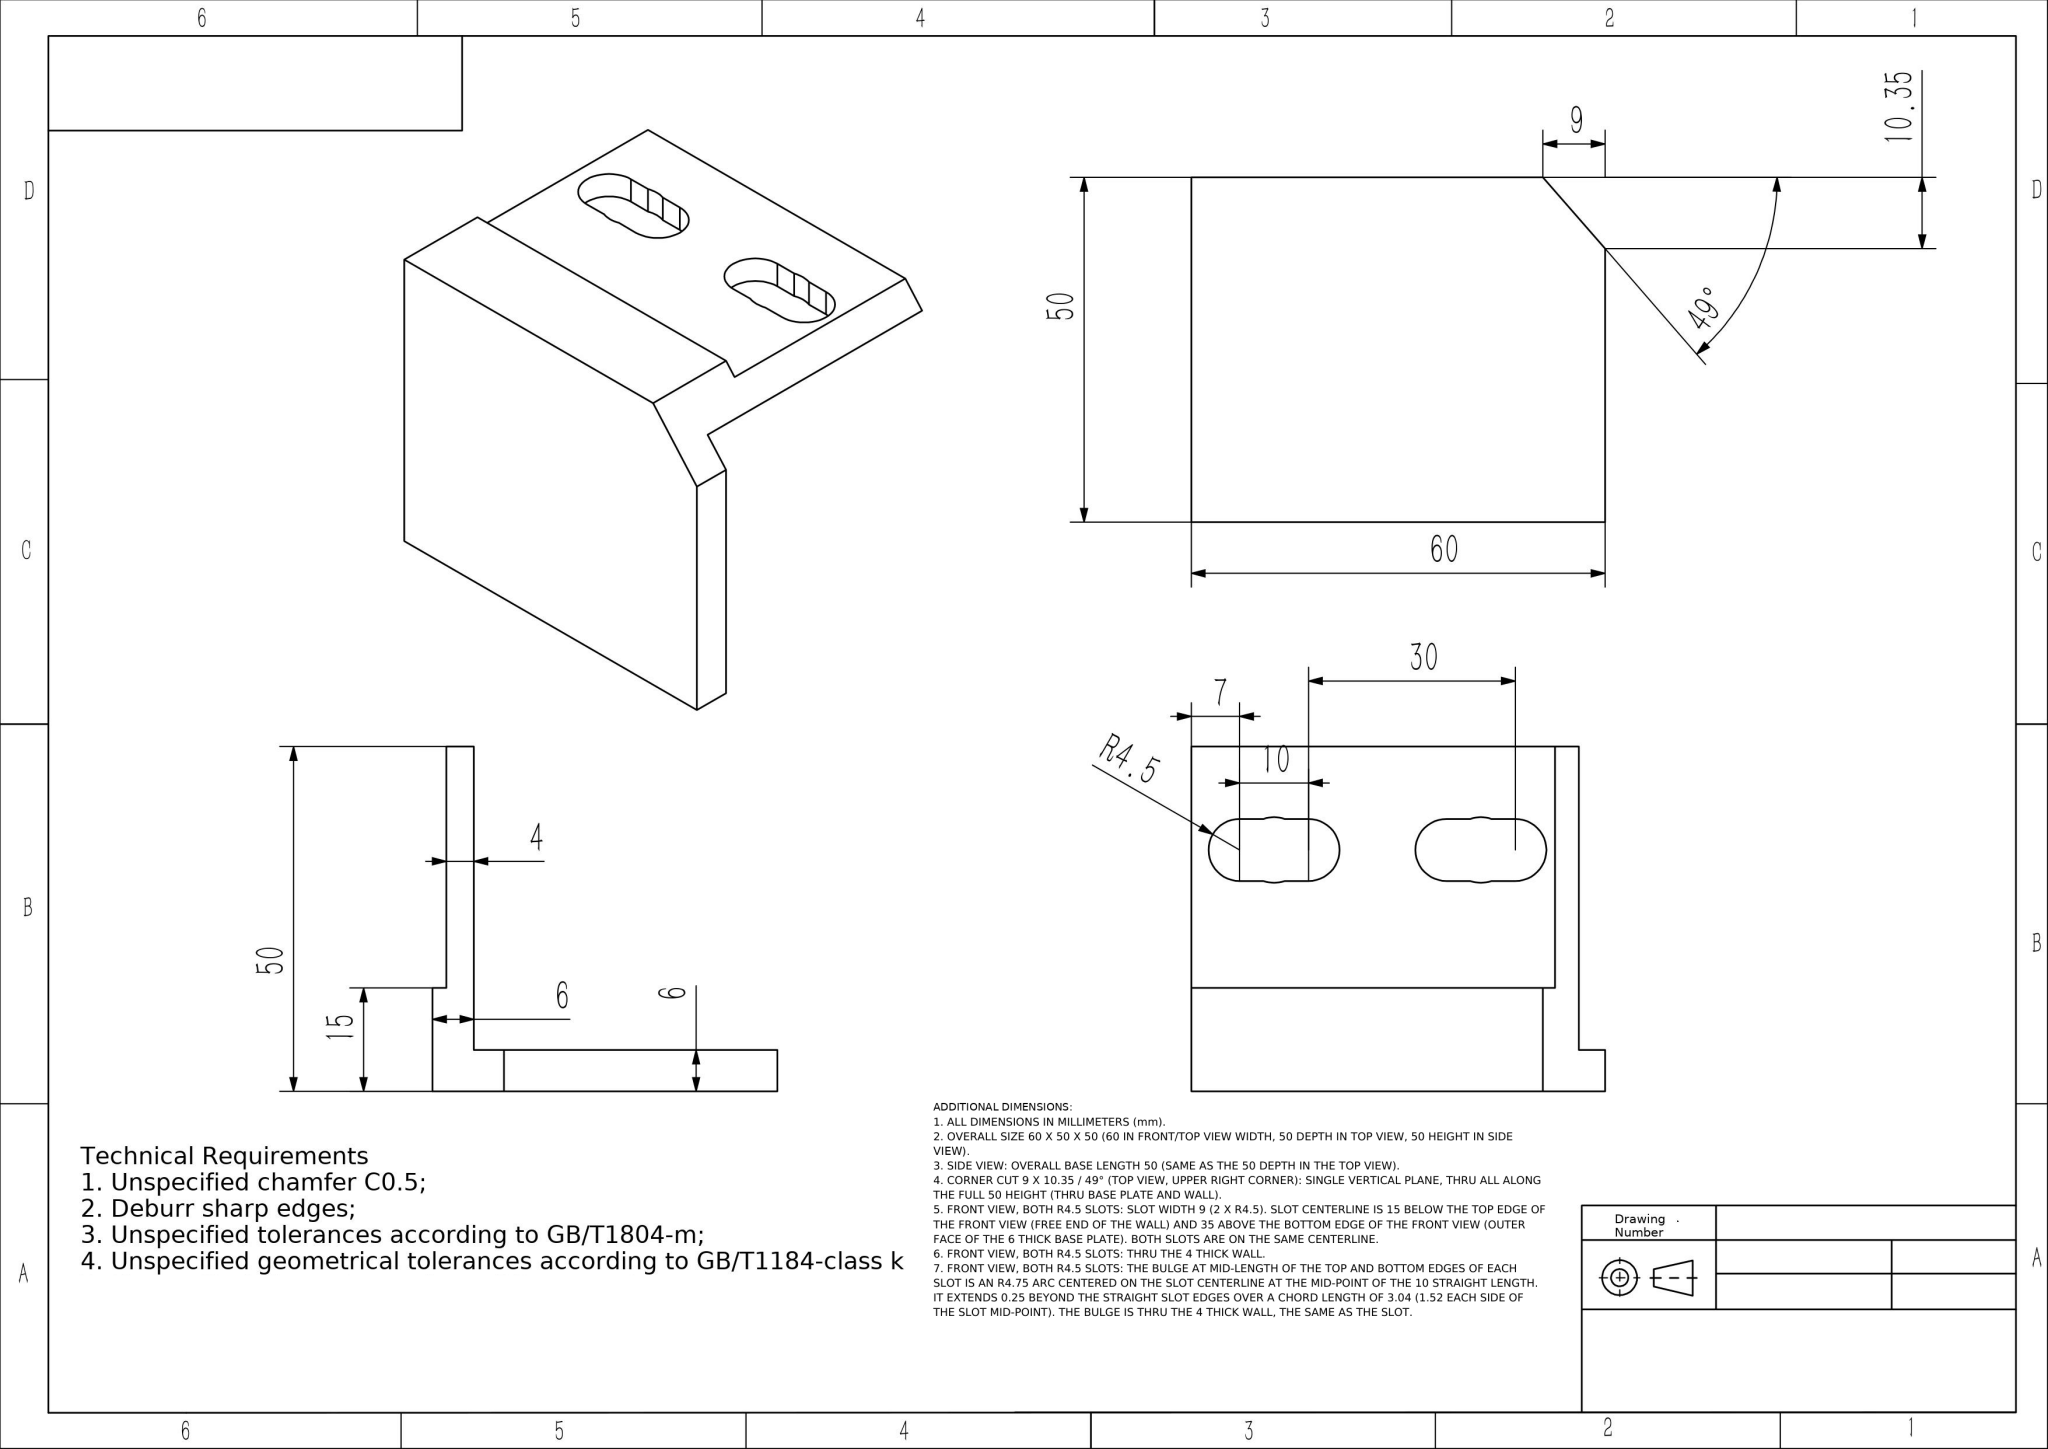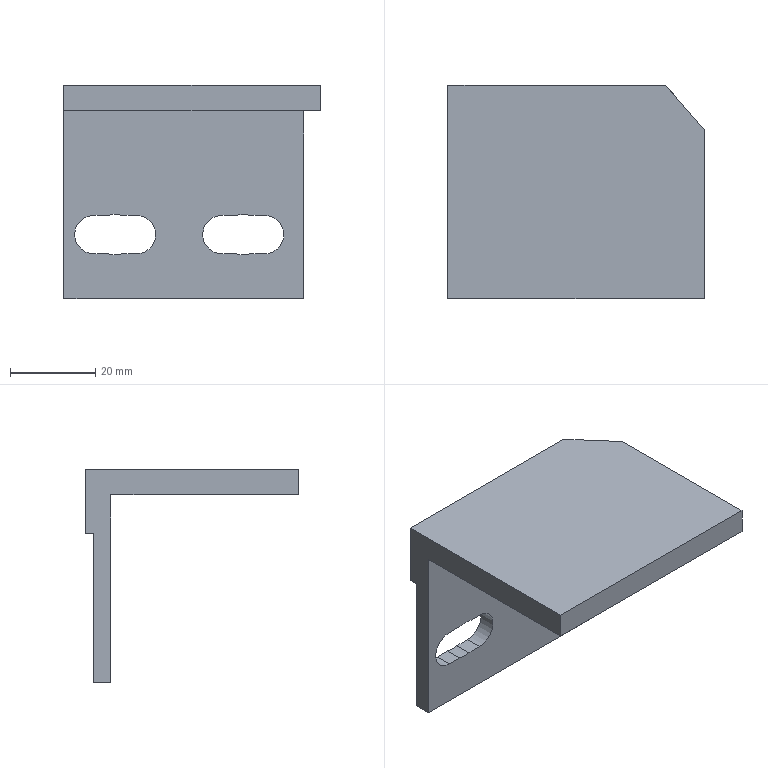Part | NX | mm | 1 solid | 29 faces | box 60 x 50 x 50 mm | volume 27005 mm3 | plane 19 | cylinder 10 | commonest cylinder face diameters 9.5 x6 9 x4
STEP:
#1=COLOUR_RGB('',1.,0.,1.);
#2=FILL_AREA_STYLE_COLOUR('',#1);
#3=FILL_AREA_STYLE('',(#2));
#4=SURFACE_STYLE_FILL_AREA(#3);
#5=SURFACE_SIDE_STYLE('',(#4));
#6=SURFACE_STYLE_USAGE(.BOTH.,#5);
#7=PRESENTATION_STYLE_ASSIGNMENT((#6));
#8=CARTESIAN_POINT('',(12.,19.,-24.25));
#9=VERTEX_POINT('',#8);
#10=CARTESIAN_POINT('',(13.521,19.,-24.5));
#11=VERTEX_POINT('',#10);
#12=CARTESIAN_POINT('',(12.,19.,-29.));
#13=DIRECTION('',(0.,1.,0.));
#14=DIRECTION('',(0.,0.,1.));
#15=AXIS2_PLACEMENT_3D('',#12,#13,#14);
#16=CIRCLE('',#15,4.75);
#17=EDGE_CURVE('',#9,#11,#16,.T.);
#18=ORIENTED_EDGE('',*,*,#17,.F.);
#19=CARTESIAN_POINT('',(12.,23.,-24.25));
#20=VERTEX_POINT('',#19);
#21=CARTESIAN_POINT('',(12.,23.,-24.25));
#22=DIRECTION('',(0.,1.,0.));
#23=VECTOR('',#22,1000.);
#24=LINE('',#21,#23);
#25=EDGE_CURVE('',#9,#20,#24,.T.);
#26=ORIENTED_EDGE('',*,*,#25,.T.);
#27=CARTESIAN_POINT('',(13.521,23.,-24.5));
#28=VERTEX_POINT('',#27);
#29=CARTESIAN_POINT('',(12.,23.,-29.));
#30=DIRECTION('',(0.,1.,0.));
#31=DIRECTION('',(0.,0.,1.));
#32=AXIS2_PLACEMENT_3D('',#29,#30,#31);
#33=CIRCLE('',#32,4.75);
#34=EDGE_CURVE('',#20,#28,#33,.T.);
#35=ORIENTED_EDGE('',*,*,#34,.T.);
#36=CARTESIAN_POINT('',(13.521,23.,-24.5));
#37=DIRECTION('',(0.,1.,0.));
#38=VECTOR('',#37,1000.);
#39=LINE('',#36,#38);
#40=EDGE_CURVE('',#11,#28,#39,.T.);
#41=ORIENTED_EDGE('',*,*,#40,.F.);
#42=EDGE_LOOP('',(#18,#26,#35,#41));
#43=FACE_OUTER_BOUND('',#42,.T.);
#44=CARTESIAN_POINT('',(12.,23.,-29.));
#45=DIRECTION('',(0.,1.,0.));
#46=DIRECTION('',(0.,0.,1.));
#47=AXIS2_PLACEMENT_3D('',#44,#45,#46);
#48=CYLINDRICAL_SURFACE('',#47,4.75);
#49=ADVANCED_FACE('',(#43),#48,.F.);
#50=CARTESIAN_POINT('',(-18.,19.,-24.25));
#51=VERTEX_POINT('',#50);
#52=CARTESIAN_POINT('',(-16.479,19.,-24.5));
#53=VERTEX_POINT('',#52);
#54=CARTESIAN_POINT('',(-18.,19.,-29.));
#55=DIRECTION('',(0.,1.,0.));
#56=DIRECTION('',(0.,0.,1.));
#57=AXIS2_PLACEMENT_3D('',#54,#55,#56);
#58=CIRCLE('',#57,4.75);
#59=EDGE_CURVE('',#51,#53,#58,.T.);
#60=ORIENTED_EDGE('',*,*,#59,.F.);
#61=CARTESIAN_POINT('',(-18.,23.,-24.25));
#62=VERTEX_POINT('',#61);
#63=CARTESIAN_POINT('',(-18.,23.,-24.25));
#64=DIRECTION('',(0.,1.,0.));
#65=VECTOR('',#64,1000.);
#66=LINE('',#63,#65);
#67=EDGE_CURVE('',#51,#62,#66,.T.);
#68=ORIENTED_EDGE('',*,*,#67,.T.);
#69=CARTESIAN_POINT('',(-16.479,23.,-24.5));
#70=VERTEX_POINT('',#69);
#71=CARTESIAN_POINT('',(-18.,23.,-29.));
#72=DIRECTION('',(0.,1.,0.));
#73=DIRECTION('',(0.,0.,1.));
#74=AXIS2_PLACEMENT_3D('',#71,#72,#73);
#75=CIRCLE('',#74,4.75);
#76=EDGE_CURVE('',#62,#70,#75,.T.);
#77=ORIENTED_EDGE('',*,*,#76,.T.);
#78=CARTESIAN_POINT('',(-16.479,23.,-24.5));
#79=DIRECTION('',(0.,1.,0.));
#80=VECTOR('',#79,1000.);
#81=LINE('',#78,#80);
#82=EDGE_CURVE('',#53,#70,#81,.T.);
#83=ORIENTED_EDGE('',*,*,#82,.F.);
#84=EDGE_LOOP('',(#60,#68,#77,#83));
#85=FACE_OUTER_BOUND('',#84,.T.);
#86=CARTESIAN_POINT('',(-18.,23.,-29.));
#87=DIRECTION('',(0.,1.,0.));
#88=DIRECTION('',(0.,0.,1.));
#89=AXIS2_PLACEMENT_3D('',#86,#87,#88);
#90=CYLINDRICAL_SURFACE('',#89,4.75);
#91=ADVANCED_FACE('',(#85),#90,.F.);
#92=CARTESIAN_POINT('',(10.479,19.,-33.5));
#93=VERTEX_POINT('',#92);
#94=CARTESIAN_POINT('',(7.,19.,-33.5));
#95=VERTEX_POINT('',#94);
#96=CARTESIAN_POINT('',(30.,19.,-33.5));
#97=DIRECTION('',(-1.,0.,0.));
#98=VECTOR('',#97,1000.);
#99=LINE('',#96,#98);
#100=EDGE_CURVE('',#93,#95,#99,.T.);
#101=ORIENTED_EDGE('',*,*,#100,.F.);
#102=CARTESIAN_POINT('',(10.479,23.,-33.5));
#103=VERTEX_POINT('',#102);
#104=CARTESIAN_POINT('',(10.479,23.,-33.5));
#105=DIRECTION('',(0.,1.,0.));
#106=VECTOR('',#105,1000.);
#107=LINE('',#104,#106);
#108=EDGE_CURVE('',#93,#103,#107,.T.);
#109=ORIENTED_EDGE('',*,*,#108,.T.);
#110=CARTESIAN_POINT('',(7.,23.,-33.5));
#111=VERTEX_POINT('',#110);
#112=CARTESIAN_POINT('',(7.,23.,-33.5));
#113=DIRECTION('',(-1.,0.,0.));
#114=VECTOR('',#113,1000.);
#115=LINE('',#112,#114);
#116=EDGE_CURVE('',#103,#111,#115,.T.);
#117=ORIENTED_EDGE('',*,*,#116,.T.);
#118=CARTESIAN_POINT('',(7.,-21.,-33.5));
#119=DIRECTION('',(0.,1.,0.));
#120=VECTOR('',#119,1000.);
#121=LINE('',#118,#120);
#122=EDGE_CURVE('',#95,#111,#121,.T.);
#123=ORIENTED_EDGE('',*,*,#122,.F.);
#124=EDGE_LOOP('',(#101,#109,#117,#123));
#125=FACE_OUTER_BOUND('',#124,.T.);
#126=CARTESIAN_POINT('',(7.,-21.,-33.5));
#127=DIRECTION('',(0.,0.,-1.));
#128=DIRECTION('',(0.,1.,0.));
#129=AXIS2_PLACEMENT_3D('',#126,#127,#128);
#130=PLANE('',#129);
#131=ADVANCED_FACE('',(#125),#130,.F.);
#132=CARTESIAN_POINT('',(-30.,23.,-9.));
#133=VERTEX_POINT('',#132);
#134=CARTESIAN_POINT('',(22.739,23.,-9.));
#135=VERTEX_POINT('',#134);
#136=CARTESIAN_POINT('',(-30.,23.,-9.));
#137=DIRECTION('',(1.,0.,0.));
#138=VECTOR('',#137,1000.);
#139=LINE('',#136,#138);
#140=EDGE_CURVE('',#133,#135,#139,.T.);
#141=ORIENTED_EDGE('',*,*,#140,.T.);
#142=CARTESIAN_POINT('',(22.739,23.,-44.));
#143=VERTEX_POINT('',#142);
#144=CARTESIAN_POINT('',(22.739,23.,-44.));
#145=DIRECTION('',(-0.,0.,-1.));
#146=VECTOR('',#145,1000.);
#147=LINE('',#144,#146);
#148=EDGE_CURVE('',#135,#143,#147,.T.);
#149=ORIENTED_EDGE('',*,*,#148,.T.);
#150=CARTESIAN_POINT('',(-30.,23.,-44.));
#151=VERTEX_POINT('',#150);
#152=CARTESIAN_POINT('',(0.,23.,-44.));
#153=DIRECTION('',(-1.,0.,0.));
#154=VECTOR('',#153,1000.);
#155=LINE('',#152,#154);
#156=EDGE_CURVE('',#143,#151,#155,.T.);
#157=ORIENTED_EDGE('',*,*,#156,.T.);
#158=CARTESIAN_POINT('',(-30.,23.,6.));
#159=DIRECTION('',(0.,0.,-1.));
#160=VECTOR('',#159,1000.);
#161=LINE('',#158,#160);
#162=EDGE_CURVE('',#133,#151,#161,.T.);
#163=ORIENTED_EDGE('',*,*,#162,.F.);
#164=EDGE_LOOP('',(#141,#149,#157,#163));
#165=FACE_OUTER_BOUND('',#164,.T.);
#166=CARTESIAN_POINT('',(-16.479,23.,-33.5));
#167=VERTEX_POINT('',#166);
#168=CARTESIAN_POINT('',(-19.521,23.,-33.5));
#169=VERTEX_POINT('',#168);
#170=CARTESIAN_POINT('',(-18.,23.,-29.));
#171=DIRECTION('',(0.,1.,0.));
#172=DIRECTION('',(0.,0.,1.));
#173=AXIS2_PLACEMENT_3D('',#170,#171,#172);
#174=CIRCLE('',#173,4.75);
#175=EDGE_CURVE('',#167,#169,#174,.T.);
#176=ORIENTED_EDGE('',*,*,#175,.F.);
#177=CARTESIAN_POINT('',(-13.,23.,-33.5));
#178=VERTEX_POINT('',#177);
#179=CARTESIAN_POINT('',(-23.,23.,-33.5));
#180=DIRECTION('',(-1.,0.,0.));
#181=VECTOR('',#180,1000.);
#182=LINE('',#179,#181);
#183=EDGE_CURVE('',#178,#167,#182,.T.);
#184=ORIENTED_EDGE('',*,*,#183,.F.);
#185=CARTESIAN_POINT('',(-13.,23.,-24.5));
#186=VERTEX_POINT('',#185);
#187=CARTESIAN_POINT('',(-13.,23.,-29.));
#188=DIRECTION('',(0.,1.,0.));
#189=DIRECTION('',(0.,0.,1.));
#190=AXIS2_PLACEMENT_3D('',#187,#188,#189);
#191=CIRCLE('',#190,4.5);
#192=EDGE_CURVE('',#186,#178,#191,.T.);
#193=ORIENTED_EDGE('',*,*,#192,.F.);
#194=CARTESIAN_POINT('',(-23.,23.,-24.5));
#195=DIRECTION('',(1.,0.,-0.));
#196=VECTOR('',#195,1000.);
#197=LINE('',#194,#196);
#198=EDGE_CURVE('',#70,#186,#197,.T.);
#199=ORIENTED_EDGE('',*,*,#198,.F.);
#200=ORIENTED_EDGE('',*,*,#76,.F.);
#201=CARTESIAN_POINT('',(-19.521,23.,-24.5));
#202=VERTEX_POINT('',#201);
#203=CARTESIAN_POINT('',(-18.,23.,-29.));
#204=DIRECTION('',(0.,1.,0.));
#205=DIRECTION('',(0.,0.,1.));
#206=AXIS2_PLACEMENT_3D('',#203,#204,#205);
#207=CIRCLE('',#206,4.75);
#208=EDGE_CURVE('',#202,#62,#207,.T.);
#209=ORIENTED_EDGE('',*,*,#208,.F.);
#210=CARTESIAN_POINT('',(-23.,23.,-24.5));
#211=VERTEX_POINT('',#210);
#212=CARTESIAN_POINT('',(-23.,23.,-24.5));
#213=DIRECTION('',(1.,0.,-0.));
#214=VECTOR('',#213,1000.);
#215=LINE('',#212,#214);
#216=EDGE_CURVE('',#211,#202,#215,.T.);
#217=ORIENTED_EDGE('',*,*,#216,.F.);
#218=CARTESIAN_POINT('',(-23.,23.,-33.5));
#219=VERTEX_POINT('',#218);
#220=CARTESIAN_POINT('',(-23.,23.,-29.));
#221=DIRECTION('',(0.,1.,0.));
#222=DIRECTION('',(0.,0.,1.));
#223=AXIS2_PLACEMENT_3D('',#220,#221,#222);
#224=CIRCLE('',#223,4.5);
#225=EDGE_CURVE('',#219,#211,#224,.T.);
#226=ORIENTED_EDGE('',*,*,#225,.F.);
#227=CARTESIAN_POINT('',(-23.,23.,-33.5));
#228=DIRECTION('',(-1.,0.,0.));
#229=VECTOR('',#228,1000.);
#230=LINE('',#227,#229);
#231=EDGE_CURVE('',#169,#219,#230,.T.);
#232=ORIENTED_EDGE('',*,*,#231,.F.);
#233=EDGE_LOOP('',(#176,#184,#193,#199,#200,#209,#217,#226,#232));
#234=FACE_BOUND('',#233,.T.);
#235=CARTESIAN_POINT('',(13.521,23.,-33.5));
#236=VERTEX_POINT('',#235);
#237=CARTESIAN_POINT('',(12.,23.,-29.));
#238=DIRECTION('',(0.,1.,0.));
#239=DIRECTION('',(0.,0.,1.));
#240=AXIS2_PLACEMENT_3D('',#237,#238,#239);
#241=CIRCLE('',#240,4.75);
#242=EDGE_CURVE('',#236,#103,#241,.T.);
#243=ORIENTED_EDGE('',*,*,#242,.F.);
#244=CARTESIAN_POINT('',(17.,23.,-33.5));
#245=VERTEX_POINT('',#244);
#246=CARTESIAN_POINT('',(7.,23.,-33.5));
#247=DIRECTION('',(-1.,0.,0.));
#248=VECTOR('',#247,1000.);
#249=LINE('',#246,#248);
#250=EDGE_CURVE('',#245,#236,#249,.T.);
#251=ORIENTED_EDGE('',*,*,#250,.F.);
#252=CARTESIAN_POINT('',(17.,23.,-24.5));
#253=VERTEX_POINT('',#252);
#254=CARTESIAN_POINT('',(17.,23.,-29.));
#255=DIRECTION('',(0.,1.,0.));
#256=DIRECTION('',(0.,0.,1.));
#257=AXIS2_PLACEMENT_3D('',#254,#255,#256);
#258=CIRCLE('',#257,4.5);
#259=EDGE_CURVE('',#253,#245,#258,.T.);
#260=ORIENTED_EDGE('',*,*,#259,.F.);
#261=CARTESIAN_POINT('',(7.,23.,-24.5));
#262=DIRECTION('',(1.,0.,-0.));
#263=VECTOR('',#262,1000.);
#264=LINE('',#261,#263);
#265=EDGE_CURVE('',#28,#253,#264,.T.);
#266=ORIENTED_EDGE('',*,*,#265,.F.);
#267=ORIENTED_EDGE('',*,*,#34,.F.);
#268=CARTESIAN_POINT('',(10.479,23.,-24.5));
#269=VERTEX_POINT('',#268);
#270=CARTESIAN_POINT('',(12.,23.,-29.));
#271=DIRECTION('',(0.,1.,0.));
#272=DIRECTION('',(0.,0.,1.));
#273=AXIS2_PLACEMENT_3D('',#270,#271,#272);
#274=CIRCLE('',#273,4.75);
#275=EDGE_CURVE('',#269,#20,#274,.T.);
#276=ORIENTED_EDGE('',*,*,#275,.F.);
#277=CARTESIAN_POINT('',(7.,23.,-24.5));
#278=VERTEX_POINT('',#277);
#279=CARTESIAN_POINT('',(7.,23.,-24.5));
#280=DIRECTION('',(1.,0.,-0.));
#281=VECTOR('',#280,1000.);
#282=LINE('',#279,#281);
#283=EDGE_CURVE('',#278,#269,#282,.T.);
#284=ORIENTED_EDGE('',*,*,#283,.F.);
#285=CARTESIAN_POINT('',(7.,23.,-29.));
#286=DIRECTION('',(0.,1.,0.));
#287=DIRECTION('',(0.,0.,1.));
#288=AXIS2_PLACEMENT_3D('',#285,#286,#287);
#289=CIRCLE('',#288,4.5);
#290=EDGE_CURVE('',#111,#278,#289,.T.);
#291=ORIENTED_EDGE('',*,*,#290,.F.);
#292=ORIENTED_EDGE('',*,*,#116,.F.);
#293=EDGE_LOOP('',(#243,#251,#260,#266,#267,#276,#284,#291,#292));
#294=FACE_BOUND('',#293,.T.);
#295=CARTESIAN_POINT('',(-30.,23.,-44.));
#296=DIRECTION('',(0.,-1.,-0.));
#297=DIRECTION('',(0.,0.,-1.));
#298=AXIS2_PLACEMENT_3D('',#295,#296,#297);
#299=PLANE('',#298);
#300=ADVANCED_FACE('',(#165,#234,#294),#299,.F.);
#301=CARTESIAN_POINT('',(17.,19.,-24.5));
#302=VERTEX_POINT('',#301);
#303=CARTESIAN_POINT('',(30.,19.,-24.5));
#304=DIRECTION('',(1.,0.,-0.));
#305=VECTOR('',#304,1000.);
#306=LINE('',#303,#305);
#307=EDGE_CURVE('',#11,#302,#306,.T.);
#308=ORIENTED_EDGE('',*,*,#307,.F.);
#309=ORIENTED_EDGE('',*,*,#40,.T.);
#310=ORIENTED_EDGE('',*,*,#265,.T.);
#311=CARTESIAN_POINT('',(17.,-21.,-24.5));
#312=DIRECTION('',(0.,1.,0.));
#313=VECTOR('',#312,1000.);
#314=LINE('',#311,#313);
#315=EDGE_CURVE('',#302,#253,#314,.T.);
#316=ORIENTED_EDGE('',*,*,#315,.F.);
#317=EDGE_LOOP('',(#308,#309,#310,#316));
#318=FACE_OUTER_BOUND('',#317,.T.);
#319=CARTESIAN_POINT('',(7.,-21.,-24.5));
#320=DIRECTION('',(0.,-0.,1.));
#321=DIRECTION('',(1.,0.,-0.));
#322=AXIS2_PLACEMENT_3D('',#319,#320,#321);
#323=PLANE('',#322);
#324=ADVANCED_FACE('',(#318),#323,.F.);
#325=CARTESIAN_POINT('',(-19.521,19.,-33.5));
#326=VERTEX_POINT('',#325);
#327=CARTESIAN_POINT('',(-23.,19.,-33.5));
#328=VERTEX_POINT('',#327);
#329=CARTESIAN_POINT('',(30.,19.,-33.5));
#330=DIRECTION('',(-1.,0.,0.));
#331=VECTOR('',#330,1000.);
#332=LINE('',#329,#331);
#333=EDGE_CURVE('',#326,#328,#332,.T.);
#334=ORIENTED_EDGE('',*,*,#333,.F.);
#335=CARTESIAN_POINT('',(-19.521,23.,-33.5));
#336=DIRECTION('',(0.,1.,0.));
#337=VECTOR('',#336,1000.);
#338=LINE('',#335,#337);
#339=EDGE_CURVE('',#326,#169,#338,.T.);
#340=ORIENTED_EDGE('',*,*,#339,.T.);
#341=ORIENTED_EDGE('',*,*,#231,.T.);
#342=CARTESIAN_POINT('',(-23.,-21.,-33.5));
#343=DIRECTION('',(0.,1.,0.));
#344=VECTOR('',#343,1000.);
#345=LINE('',#342,#344);
#346=EDGE_CURVE('',#328,#219,#345,.T.);
#347=ORIENTED_EDGE('',*,*,#346,.F.);
#348=EDGE_LOOP('',(#334,#340,#341,#347));
#349=FACE_OUTER_BOUND('',#348,.T.);
#350=CARTESIAN_POINT('',(-23.,-21.,-33.5));
#351=DIRECTION('',(0.,0.,-1.));
#352=DIRECTION('',(0.,1.,0.));
#353=AXIS2_PLACEMENT_3D('',#350,#351,#352);
#354=PLANE('',#353);
#355=ADVANCED_FACE('',(#349),#354,.F.);
#356=CARTESIAN_POINT('',(-13.,19.,-24.5));
#357=VERTEX_POINT('',#356);
#358=CARTESIAN_POINT('',(30.,19.,-24.5));
#359=DIRECTION('',(1.,0.,-0.));
#360=VECTOR('',#359,1000.);
#361=LINE('',#358,#360);
#362=EDGE_CURVE('',#53,#357,#361,.T.);
#363=ORIENTED_EDGE('',*,*,#362,.F.);
#364=ORIENTED_EDGE('',*,*,#82,.T.);
#365=ORIENTED_EDGE('',*,*,#198,.T.);
#366=CARTESIAN_POINT('',(-13.,-21.,-24.5));
#367=DIRECTION('',(0.,1.,0.));
#368=VECTOR('',#367,1000.);
#369=LINE('',#366,#368);
#370=EDGE_CURVE('',#357,#186,#369,.T.);
#371=ORIENTED_EDGE('',*,*,#370,.F.);
#372=EDGE_LOOP('',(#363,#364,#365,#371));
#373=FACE_OUTER_BOUND('',#372,.T.);
#374=CARTESIAN_POINT('',(-23.,-21.,-24.5));
#375=DIRECTION('',(0.,-0.,1.));
#376=DIRECTION('',(1.,0.,-0.));
#377=AXIS2_PLACEMENT_3D('',#374,#375,#376);
#378=PLANE('',#377);
#379=ADVANCED_FACE('',(#373),#378,.F.);
#380=CARTESIAN_POINT('',(30.,-25.,0.));
#381=VERTEX_POINT('',#380);
#382=CARTESIAN_POINT('',(30.,14.647,0.));
#383=VERTEX_POINT('',#382);
#384=CARTESIAN_POINT('',(30.,-25.,0.));
#385=DIRECTION('',(0.,1.,0.));
#386=VECTOR('',#385,1000.);
#387=LINE('',#384,#386);
#388=EDGE_CURVE('',#381,#383,#387,.T.);
#389=ORIENTED_EDGE('',*,*,#388,.T.);
#390=CARTESIAN_POINT('',(30.,14.647,6.));
#391=VERTEX_POINT('',#390);
#392=CARTESIAN_POINT('',(30.,14.647,-44.));
#393=DIRECTION('',(0.,0.,1.));
#394=VECTOR('',#393,1000.);
#395=LINE('',#392,#394);
#396=EDGE_CURVE('',#383,#391,#395,.T.);
#397=ORIENTED_EDGE('',*,*,#396,.T.);
#398=CARTESIAN_POINT('',(30.,-25.,6.));
#399=VERTEX_POINT('',#398);
#400=CARTESIAN_POINT('',(30.,-25.,6.));
#401=DIRECTION('',(0.,1.,0.));
#402=VECTOR('',#401,1000.);
#403=LINE('',#400,#402);
#404=EDGE_CURVE('',#399,#391,#403,.T.);
#405=ORIENTED_EDGE('',*,*,#404,.F.);
#406=CARTESIAN_POINT('',(30.,-25.,6.));
#407=DIRECTION('',(0.,0.,-1.));
#408=VECTOR('',#407,1000.);
#409=LINE('',#406,#408);
#410=EDGE_CURVE('',#399,#381,#409,.T.);
#411=ORIENTED_EDGE('',*,*,#410,.T.);
#412=EDGE_LOOP('',(#389,#397,#405,#411));
#413=FACE_OUTER_BOUND('',#412,.T.);
#414=CARTESIAN_POINT('',(30.,-25.,6.));
#415=DIRECTION('',(-1.,0.,0.));
#416=DIRECTION('',(0.,0.,1.));
#417=AXIS2_PLACEMENT_3D('',#414,#415,#416);
#418=PLANE('',#417);
#419=ADVANCED_FACE('',(#413),#418,.F.);
#420=CARTESIAN_POINT('',(21.,25.,6.));
#421=VERTEX_POINT('',#420);
#422=CARTESIAN_POINT('',(-30.,25.,6.));
#423=VERTEX_POINT('',#422);
#424=CARTESIAN_POINT('',(-30.,25.,6.));
#425=DIRECTION('',(-1.,0.,0.));
#426=VECTOR('',#425,1000.);
#427=LINE('',#424,#426);
#428=EDGE_CURVE('',#421,#423,#427,.T.);
#429=ORIENTED_EDGE('',*,*,#428,.F.);
#430=CARTESIAN_POINT('',(21.,25.,-9.));
#431=VERTEX_POINT('',#430);
#432=CARTESIAN_POINT('',(21.,25.,-44.));
#433=DIRECTION('',(0.,0.,1.));
#434=VECTOR('',#433,1000.);
#435=LINE('',#432,#434);
#436=EDGE_CURVE('',#431,#421,#435,.T.);
#437=ORIENTED_EDGE('',*,*,#436,.F.);
#438=CARTESIAN_POINT('',(-30.,25.,-9.));
#439=VERTEX_POINT('',#438);
#440=CARTESIAN_POINT('',(-30.,25.,-9.));
#441=DIRECTION('',(1.,0.,0.));
#442=VECTOR('',#441,1000.);
#443=LINE('',#440,#442);
#444=EDGE_CURVE('',#439,#431,#443,.T.);
#445=ORIENTED_EDGE('',*,*,#444,.F.);
#446=CARTESIAN_POINT('',(-30.,25.,6.));
#447=DIRECTION('',(0.,0.,-1.));
#448=VECTOR('',#447,1000.);
#449=LINE('',#446,#448);
#450=EDGE_CURVE('',#423,#439,#449,.T.);
#451=ORIENTED_EDGE('',*,*,#450,.F.);
#452=EDGE_LOOP('',(#429,#437,#445,#451));
#453=FACE_OUTER_BOUND('',#452,.T.);
#454=CARTESIAN_POINT('',(-30.,25.,6.));
#455=DIRECTION('',(0.,-1.,0.));
#456=DIRECTION('',(0.,0.,-1.));
#457=AXIS2_PLACEMENT_3D('',#454,#455,#456);
#458=PLANE('',#457);
#459=ADVANCED_FACE('',(#453),#458,.F.);
#460=CARTESIAN_POINT('',(-30.,-25.,-9.));
#461=DIRECTION('',(0.,-1.,0.));
#462=VECTOR('',#461,1000.);
#463=LINE('',#460,#462);
#464=EDGE_CURVE('',#439,#133,#463,.T.);
#465=ORIENTED_EDGE('',*,*,#464,.T.);
#466=ORIENTED_EDGE('',*,*,#162,.T.);
#467=CARTESIAN_POINT('',(-30.,19.,-44.));
#468=VERTEX_POINT('',#467);
#469=CARTESIAN_POINT('',(-30.,25.,-44.));
#470=DIRECTION('',(0.,1.,0.));
#471=VECTOR('',#470,1000.);
#472=LINE('',#469,#471);
#473=EDGE_CURVE('',#468,#151,#472,.T.);
#474=ORIENTED_EDGE('',*,*,#473,.F.);
#475=CARTESIAN_POINT('',(-30.,19.,0.));
#476=VERTEX_POINT('',#475);
#477=CARTESIAN_POINT('',(-30.,19.,-44.));
#478=DIRECTION('',(0.,0.,1.));
#479=VECTOR('',#478,1000.);
#480=LINE('',#477,#479);
#481=EDGE_CURVE('',#468,#476,#480,.T.);
#482=ORIENTED_EDGE('',*,*,#481,.T.);
#483=CARTESIAN_POINT('',(-30.,-25.,0.));
#484=VERTEX_POINT('',#483);
#485=CARTESIAN_POINT('',(-30.,-25.,0.));
#486=DIRECTION('',(0.,-1.,0.));
#487=VECTOR('',#486,1000.);
#488=LINE('',#485,#487);
#489=EDGE_CURVE('',#476,#484,#488,.T.);
#490=ORIENTED_EDGE('',*,*,#489,.T.);
#491=CARTESIAN_POINT('',(-30.,-25.,6.));
#492=VERTEX_POINT('',#491);
#493=CARTESIAN_POINT('',(-30.,-25.,6.));
#494=DIRECTION('',(0.,0.,-1.));
#495=VECTOR('',#494,1000.);
#496=LINE('',#493,#495);
#497=EDGE_CURVE('',#492,#484,#496,.T.);
#498=ORIENTED_EDGE('',*,*,#497,.F.);
#499=CARTESIAN_POINT('',(-30.,-25.,6.));
#500=DIRECTION('',(0.,-1.,0.));
#501=VECTOR('',#500,1000.);
#502=LINE('',#499,#501);
#503=EDGE_CURVE('',#423,#492,#502,.T.);
#504=ORIENTED_EDGE('',*,*,#503,.F.);
#505=ORIENTED_EDGE('',*,*,#450,.T.);
#506=EDGE_LOOP('',(#465,#466,#474,#482,#490,#498,#504,#505));
#507=FACE_OUTER_BOUND('',#506,.T.);
#508=CARTESIAN_POINT('',(-30.,-25.,6.));
#509=DIRECTION('',(1.,0.,0.));
#510=DIRECTION('',(0.,0.,-1.));
#511=AXIS2_PLACEMENT_3D('',#508,#509,#510);
#512=PLANE('',#511);
#513=ADVANCED_FACE('',(#507),#512,.F.);
#514=CARTESIAN_POINT('',(-30.,-25.,0.));
#515=DIRECTION('',(1.,0.,0.));
#516=VECTOR('',#515,1000.);
#517=LINE('',#514,#516);
#518=EDGE_CURVE('',#484,#381,#517,.T.);
#519=ORIENTED_EDGE('',*,*,#518,.T.);
#520=ORIENTED_EDGE('',*,*,#410,.F.);
#521=CARTESIAN_POINT('',(-30.,-25.,6.));
#522=DIRECTION('',(1.,0.,0.));
#523=VECTOR('',#522,1000.);
#524=LINE('',#521,#523);
#525=EDGE_CURVE('',#492,#399,#524,.T.);
#526=ORIENTED_EDGE('',*,*,#525,.F.);
#527=ORIENTED_EDGE('',*,*,#497,.T.);
#528=EDGE_LOOP('',(#519,#520,#526,#527));
#529=FACE_OUTER_BOUND('',#528,.T.);
#530=CARTESIAN_POINT('',(-30.,-25.,6.));
#531=DIRECTION('',(0.,1.,0.));
#532=DIRECTION('',(0.,0.,1.));
#533=AXIS2_PLACEMENT_3D('',#530,#531,#532);
#534=PLANE('',#533);
#535=ADVANCED_FACE('',(#529),#534,.F.);
#536=ORIENTED_EDGE('',*,*,#404,.T.);
#537=CARTESIAN_POINT('',(21.,25.,6.));
#538=DIRECTION('',(0.6561,-0.7547,0.));
#539=VECTOR('',#538,1000.);
#540=LINE('',#537,#539);
#541=EDGE_CURVE('',#421,#391,#540,.T.);
#542=ORIENTED_EDGE('',*,*,#541,.F.);
#543=ORIENTED_EDGE('',*,*,#428,.T.);
#544=ORIENTED_EDGE('',*,*,#503,.T.);
#545=ORIENTED_EDGE('',*,*,#525,.T.);
#546=EDGE_LOOP('',(#536,#542,#543,#544,#545));
#547=FACE_OUTER_BOUND('',#546,.T.);
#548=CARTESIAN_POINT('',(0.,0.,6.));
#549=DIRECTION('',(0.,0.,-1.));
#550=DIRECTION('',(-1.,0.,0.));
#551=AXIS2_PLACEMENT_3D('',#548,#549,#550);
#552=PLANE('',#551);
#553=ADVANCED_FACE('',(#547),#552,.F.);
#554=CARTESIAN_POINT('',(26.216,19.,0.));
#555=VERTEX_POINT('',#554);
#556=CARTESIAN_POINT('',(24.34,21.158,0.));
#557=DIRECTION('',(-0.6561,0.7547,0.));
#558=VECTOR('',#557,1000.);
#559=LINE('',#556,#558);
#560=EDGE_CURVE('',#383,#555,#559,.T.);
#561=ORIENTED_EDGE('',*,*,#560,.F.);
#562=ORIENTED_EDGE('',*,*,#388,.F.);
#563=ORIENTED_EDGE('',*,*,#518,.F.);
#564=ORIENTED_EDGE('',*,*,#489,.F.);
#565=CARTESIAN_POINT('',(30.,19.,0.));
#566=DIRECTION('',(-1.,0.,0.));
#567=VECTOR('',#566,1000.);
#568=LINE('',#565,#567);
#569=EDGE_CURVE('',#555,#476,#568,.T.);
#570=ORIENTED_EDGE('',*,*,#569,.F.);
#571=EDGE_LOOP('',(#561,#562,#563,#564,#570));
#572=FACE_OUTER_BOUND('',#571,.T.);
#573=CARTESIAN_POINT('',(0.,0.,0.));
#574=DIRECTION('',(0.,0.,-1.));
#575=DIRECTION('',(-1.,0.,0.));
#576=AXIS2_PLACEMENT_3D('',#573,#574,#575);
#577=PLANE('',#576);
#578=ADVANCED_FACE('',(#572),#577,.T.);
#579=CARTESIAN_POINT('',(17.,19.,-33.5));
#580=VERTEX_POINT('',#579);
#581=CARTESIAN_POINT('',(13.521,19.,-33.5));
#582=VERTEX_POINT('',#581);
#583=CARTESIAN_POINT('',(30.,19.,-33.5));
#584=DIRECTION('',(-1.,0.,0.));
#585=VECTOR('',#584,1000.);
#586=LINE('',#583,#585);
#587=EDGE_CURVE('',#580,#582,#586,.T.);
#588=ORIENTED_EDGE('',*,*,#587,.T.);
#589=CARTESIAN_POINT('',(12.,19.,-29.));
#590=DIRECTION('',(0.,1.,0.));
#591=DIRECTION('',(0.,0.,1.));
#592=AXIS2_PLACEMENT_3D('',#589,#590,#591);
#593=CIRCLE('',#592,4.75);
#594=EDGE_CURVE('',#582,#93,#593,.T.);
#595=ORIENTED_EDGE('',*,*,#594,.T.);
#596=ORIENTED_EDGE('',*,*,#100,.T.);
#597=CARTESIAN_POINT('',(7.,19.,-24.5));
#598=VERTEX_POINT('',#597);
#599=CARTESIAN_POINT('',(7.,19.,-29.));
#600=DIRECTION('',(0.,1.,0.));
#601=DIRECTION('',(0.,0.,1.));
#602=AXIS2_PLACEMENT_3D('',#599,#600,#601);
#603=CIRCLE('',#602,4.5);
#604=EDGE_CURVE('',#95,#598,#603,.T.);
#605=ORIENTED_EDGE('',*,*,#604,.T.);
#606=CARTESIAN_POINT('',(10.479,19.,-24.5));
#607=VERTEX_POINT('',#606);
#608=CARTESIAN_POINT('',(30.,19.,-24.5));
#609=DIRECTION('',(1.,0.,-0.));
#610=VECTOR('',#609,1000.);
#611=LINE('',#608,#610);
#612=EDGE_CURVE('',#598,#607,#611,.T.);
#613=ORIENTED_EDGE('',*,*,#612,.T.);
#614=CARTESIAN_POINT('',(12.,19.,-29.));
#615=DIRECTION('',(0.,1.,0.));
#616=DIRECTION('',(0.,0.,1.));
#617=AXIS2_PLACEMENT_3D('',#614,#615,#616);
#618=CIRCLE('',#617,4.75);
#619=EDGE_CURVE('',#607,#9,#618,.T.);
#620=ORIENTED_EDGE('',*,*,#619,.T.);
#621=ORIENTED_EDGE('',*,*,#17,.T.);
#622=ORIENTED_EDGE('',*,*,#307,.T.);
#623=CARTESIAN_POINT('',(17.,19.,-29.));
#624=DIRECTION('',(0.,1.,0.));
#625=DIRECTION('',(0.,0.,1.));
#626=AXIS2_PLACEMENT_3D('',#623,#624,#625);
#627=CIRCLE('',#626,4.5);
#628=EDGE_CURVE('',#302,#580,#627,.T.);
#629=ORIENTED_EDGE('',*,*,#628,.T.);
#630=EDGE_LOOP('',(#588,#595,#596,#605,#613,#620,#621,#622,#629));
#631=FACE_BOUND('',#630,.T.);
#632=CARTESIAN_POINT('',(-13.,19.,-33.5));
#633=VERTEX_POINT('',#632);
#634=CARTESIAN_POINT('',(-16.479,19.,-33.5));
#635=VERTEX_POINT('',#634);
#636=CARTESIAN_POINT('',(30.,19.,-33.5));
#637=DIRECTION('',(-1.,0.,0.));
#638=VECTOR('',#637,1000.);
#639=LINE('',#636,#638);
#640=EDGE_CURVE('',#633,#635,#639,.T.);
#641=ORIENTED_EDGE('',*,*,#640,.T.);
#642=CARTESIAN_POINT('',(-18.,19.,-29.));
#643=DIRECTION('',(0.,1.,0.));
#644=DIRECTION('',(0.,0.,1.));
#645=AXIS2_PLACEMENT_3D('',#642,#643,#644);
#646=CIRCLE('',#645,4.75);
#647=EDGE_CURVE('',#635,#326,#646,.T.);
#648=ORIENTED_EDGE('',*,*,#647,.T.);
#649=ORIENTED_EDGE('',*,*,#333,.T.);
#650=CARTESIAN_POINT('',(-23.,19.,-24.5));
#651=VERTEX_POINT('',#650);
#652=CARTESIAN_POINT('',(-23.,19.,-29.));
#653=DIRECTION('',(0.,1.,0.));
#654=DIRECTION('',(0.,0.,1.));
#655=AXIS2_PLACEMENT_3D('',#652,#653,#654);
#656=CIRCLE('',#655,4.5);
#657=EDGE_CURVE('',#328,#651,#656,.T.);
#658=ORIENTED_EDGE('',*,*,#657,.T.);
#659=CARTESIAN_POINT('',(-19.521,19.,-24.5));
#660=VERTEX_POINT('',#659);
#661=CARTESIAN_POINT('',(30.,19.,-24.5));
#662=DIRECTION('',(1.,0.,-0.));
#663=VECTOR('',#662,1000.);
#664=LINE('',#661,#663);
#665=EDGE_CURVE('',#651,#660,#664,.T.);
#666=ORIENTED_EDGE('',*,*,#665,.T.);
#667=CARTESIAN_POINT('',(-18.,19.,-29.));
#668=DIRECTION('',(0.,1.,0.));
#669=DIRECTION('',(0.,0.,1.));
#670=AXIS2_PLACEMENT_3D('',#667,#668,#669);
#671=CIRCLE('',#670,4.75);
#672=EDGE_CURVE('',#660,#51,#671,.T.);
#673=ORIENTED_EDGE('',*,*,#672,.T.);
#674=ORIENTED_EDGE('',*,*,#59,.T.);
#675=ORIENTED_EDGE('',*,*,#362,.T.);
#676=CARTESIAN_POINT('',(-13.,19.,-29.));
#677=DIRECTION('',(0.,1.,0.));
#678=DIRECTION('',(0.,0.,1.));
#679=AXIS2_PLACEMENT_3D('',#676,#677,#678);
#680=CIRCLE('',#679,4.5);
#681=EDGE_CURVE('',#357,#633,#680,.T.);
#682=ORIENTED_EDGE('',*,*,#681,.T.);
#683=EDGE_LOOP('',(#641,#648,#649,#658,#666,#673,#674,#675,#682));
#684=FACE_BOUND('',#683,.T.);
#685=CARTESIAN_POINT('',(26.216,19.,-44.));
#686=VERTEX_POINT('',#685);
#687=CARTESIAN_POINT('',(30.,19.,-44.));
#688=DIRECTION('',(-1.,0.,0.));
#689=VECTOR('',#688,1000.);
#690=LINE('',#687,#689);
#691=EDGE_CURVE('',#686,#468,#690,.T.);
#692=ORIENTED_EDGE('',*,*,#691,.F.);
#693=CARTESIAN_POINT('',(26.216,19.,-44.));
#694=DIRECTION('',(0.,0.,1.));
#695=VECTOR('',#694,1000.);
#696=LINE('',#693,#695);
#697=EDGE_CURVE('',#686,#555,#696,.T.);
#698=ORIENTED_EDGE('',*,*,#697,.T.);
#699=ORIENTED_EDGE('',*,*,#569,.T.);
#700=ORIENTED_EDGE('',*,*,#481,.F.);
#701=EDGE_LOOP('',(#692,#698,#699,#700));
#702=FACE_OUTER_BOUND('',#701,.T.);
#703=CARTESIAN_POINT('',(30.,19.,-44.));
#704=DIRECTION('',(0.,1.,0.));
#705=DIRECTION('',(0.,0.,1.));
#706=AXIS2_PLACEMENT_3D('',#703,#704,#705);
#707=PLANE('',#706);
#708=ADVANCED_FACE('',(#631,#684,#702),#707,.F.);
#709=CARTESIAN_POINT('',(24.34,21.158,-44.));
#710=DIRECTION('',(-0.6561,0.7547,0.));
#711=VECTOR('',#710,1000.);
#712=LINE('',#709,#711);
#713=EDGE_CURVE('',#686,#143,#712,.T.);
#714=ORIENTED_EDGE('',*,*,#713,.F.);
#715=ORIENTED_EDGE('',*,*,#691,.T.);
#716=ORIENTED_EDGE('',*,*,#473,.T.);
#717=ORIENTED_EDGE('',*,*,#156,.F.);
#718=EDGE_LOOP('',(#714,#715,#716,#717));
#719=FACE_OUTER_BOUND('',#718,.T.);
#720=CARTESIAN_POINT('',(0.,0.,-44.));
#721=DIRECTION('',(0.,0.,-1.));
#722=DIRECTION('',(-1.,0.,0.));
#723=AXIS2_PLACEMENT_3D('',#720,#721,#722);
#724=PLANE('',#723);
#725=ADVANCED_FACE('',(#719),#724,.T.);
#726=ORIENTED_EDGE('',*,*,#444,.T.);
#727=CARTESIAN_POINT('',(-0.9511,50.252,-9.));
#728=DIRECTION('',(0.6561,-0.7547,0.));
#729=VECTOR('',#728,1000.);
#730=LINE('',#727,#729);
#731=EDGE_CURVE('',#431,#135,#730,.T.);
#732=ORIENTED_EDGE('',*,*,#731,.T.);
#733=ORIENTED_EDGE('',*,*,#140,.F.);
#734=ORIENTED_EDGE('',*,*,#464,.F.);
#735=EDGE_LOOP('',(#726,#732,#733,#734));
#736=FACE_OUTER_BOUND('',#735,.T.);
#737=CARTESIAN_POINT('',(-30.,25.,-9.));
#738=DIRECTION('',(0.,0.,1.));
#739=DIRECTION('',(1.,0.,0.));
#740=AXIS2_PLACEMENT_3D('',#737,#738,#739);
#741=PLANE('',#740);
#742=ADVANCED_FACE('',(#736),#741,.F.);
#743=ORIENTED_EDGE('',*,*,#560,.T.);
#744=ORIENTED_EDGE('',*,*,#697,.F.);
#745=ORIENTED_EDGE('',*,*,#713,.T.);
#746=ORIENTED_EDGE('',*,*,#148,.F.);
#747=ORIENTED_EDGE('',*,*,#731,.F.);
#748=ORIENTED_EDGE('',*,*,#436,.T.);
#749=ORIENTED_EDGE('',*,*,#541,.T.);
#750=ORIENTED_EDGE('',*,*,#396,.F.);
#751=EDGE_LOOP('',(#743,#744,#745,#746,#747,#748,#749,#750));
#752=FACE_OUTER_BOUND('',#751,.T.);
#753=CARTESIAN_POINT('',(21.,25.,-44.));
#754=DIRECTION('',(-0.7547,-0.6561,0.));
#755=DIRECTION('',(0.6561,-0.7547,0.));
#756=AXIS2_PLACEMENT_3D('',#753,#754,#755);
#757=PLANE('',#756);
#758=ADVANCED_FACE('',(#752),#757,.F.);
#759=ORIENTED_EDGE('',*,*,#346,.T.);
#760=ORIENTED_EDGE('',*,*,#225,.T.);
#761=CARTESIAN_POINT('',(-23.,-21.,-24.5));
#762=DIRECTION('',(0.,1.,0.));
#763=VECTOR('',#762,1000.);
#764=LINE('',#761,#763);
#765=EDGE_CURVE('',#651,#211,#764,.T.);
#766=ORIENTED_EDGE('',*,*,#765,.F.);
#767=ORIENTED_EDGE('',*,*,#657,.F.);
#768=EDGE_LOOP('',(#759,#760,#766,#767));
#769=FACE_OUTER_BOUND('',#768,.T.);
#770=CARTESIAN_POINT('',(-23.,-21.,-29.));
#771=DIRECTION('',(0.,1.,0.));
#772=DIRECTION('',(0.,0.,1.));
#773=AXIS2_PLACEMENT_3D('',#770,#771,#772);
#774=CYLINDRICAL_SURFACE('',#773,4.5);
#775=ADVANCED_FACE('',(#769),#774,.F.);
#776=ORIENTED_EDGE('',*,*,#183,.T.);
#777=CARTESIAN_POINT('',(-16.479,23.,-33.5));
#778=DIRECTION('',(0.,-1.,-0.));
#779=VECTOR('',#778,1000.);
#780=LINE('',#777,#779);
#781=EDGE_CURVE('',#167,#635,#780,.T.);
#782=ORIENTED_EDGE('',*,*,#781,.T.);
#783=ORIENTED_EDGE('',*,*,#640,.F.);
#784=CARTESIAN_POINT('',(-13.,-21.,-33.5));
#785=DIRECTION('',(0.,1.,0.));
#786=VECTOR('',#785,1000.);
#787=LINE('',#784,#786);
#788=EDGE_CURVE('',#633,#178,#787,.T.);
#789=ORIENTED_EDGE('',*,*,#788,.T.);
#790=EDGE_LOOP('',(#776,#782,#783,#789));
#791=FACE_OUTER_BOUND('',#790,.T.);
#792=CARTESIAN_POINT('',(-23.,-21.,-33.5));
#793=DIRECTION('',(0.,0.,-1.));
#794=DIRECTION('',(0.,1.,0.));
#795=AXIS2_PLACEMENT_3D('',#792,#793,#794);
#796=PLANE('',#795);
#797=ADVANCED_FACE('',(#791),#796,.F.);
#798=ORIENTED_EDGE('',*,*,#370,.T.);
#799=ORIENTED_EDGE('',*,*,#192,.T.);
#800=ORIENTED_EDGE('',*,*,#788,.F.);
#801=ORIENTED_EDGE('',*,*,#681,.F.);
#802=EDGE_LOOP('',(#798,#799,#800,#801));
#803=FACE_OUTER_BOUND('',#802,.T.);
#804=CARTESIAN_POINT('',(-13.,-21.,-29.));
#805=DIRECTION('',(0.,1.,0.));
#806=DIRECTION('',(0.,0.,1.));
#807=AXIS2_PLACEMENT_3D('',#804,#805,#806);
#808=CYLINDRICAL_SURFACE('',#807,4.5);
#809=ADVANCED_FACE('',(#803),#808,.F.);
#810=ORIENTED_EDGE('',*,*,#216,.T.);
#811=CARTESIAN_POINT('',(-19.521,23.,-24.5));
#812=DIRECTION('',(0.,-1.,-0.));
#813=VECTOR('',#812,1000.);
#814=LINE('',#811,#813);
#815=EDGE_CURVE('',#202,#660,#814,.T.);
#816=ORIENTED_EDGE('',*,*,#815,.T.);
#817=ORIENTED_EDGE('',*,*,#665,.F.);
#818=ORIENTED_EDGE('',*,*,#765,.T.);
#819=EDGE_LOOP('',(#810,#816,#817,#818));
#820=FACE_OUTER_BOUND('',#819,.T.);
#821=CARTESIAN_POINT('',(-23.,-21.,-24.5));
#822=DIRECTION('',(0.,-0.,1.));
#823=DIRECTION('',(1.,0.,-0.));
#824=AXIS2_PLACEMENT_3D('',#821,#822,#823);
#825=PLANE('',#824);
#826=ADVANCED_FACE('',(#820),#825,.F.);
#827=ORIENTED_EDGE('',*,*,#67,.F.);
#828=ORIENTED_EDGE('',*,*,#672,.F.);
#829=ORIENTED_EDGE('',*,*,#815,.F.);
#830=ORIENTED_EDGE('',*,*,#208,.T.);
#831=EDGE_LOOP('',(#827,#828,#829,#830));
#832=FACE_OUTER_BOUND('',#831,.T.);
#833=CARTESIAN_POINT('',(-18.,23.,-29.));
#834=DIRECTION('',(0.,1.,0.));
#835=DIRECTION('',(0.,0.,1.));
#836=AXIS2_PLACEMENT_3D('',#833,#834,#835);
#837=CYLINDRICAL_SURFACE('',#836,4.75);
#838=ADVANCED_FACE('',(#832),#837,.F.);
#839=ORIENTED_EDGE('',*,*,#647,.F.);
#840=ORIENTED_EDGE('',*,*,#781,.F.);
#841=ORIENTED_EDGE('',*,*,#175,.T.);
#842=ORIENTED_EDGE('',*,*,#339,.F.);
#843=EDGE_LOOP('',(#839,#840,#841,#842));
#844=FACE_OUTER_BOUND('',#843,.T.);
#845=CARTESIAN_POINT('',(-18.,23.,-29.));
#846=DIRECTION('',(0.,1.,0.));
#847=DIRECTION('',(0.,0.,1.));
#848=AXIS2_PLACEMENT_3D('',#845,#846,#847);
#849=CYLINDRICAL_SURFACE('',#848,4.75);
#850=ADVANCED_FACE('',(#844),#849,.F.);
#851=ORIENTED_EDGE('',*,*,#122,.T.);
#852=ORIENTED_EDGE('',*,*,#290,.T.);
#853=CARTESIAN_POINT('',(7.,-21.,-24.5));
#854=DIRECTION('',(0.,1.,0.));
#855=VECTOR('',#854,1000.);
#856=LINE('',#853,#855);
#857=EDGE_CURVE('',#598,#278,#856,.T.);
#858=ORIENTED_EDGE('',*,*,#857,.F.);
#859=ORIENTED_EDGE('',*,*,#604,.F.);
#860=EDGE_LOOP('',(#851,#852,#858,#859));
#861=FACE_OUTER_BOUND('',#860,.T.);
#862=CARTESIAN_POINT('',(7.,-21.,-29.));
#863=DIRECTION('',(0.,1.,0.));
#864=DIRECTION('',(0.,0.,1.));
#865=AXIS2_PLACEMENT_3D('',#862,#863,#864);
#866=CYLINDRICAL_SURFACE('',#865,4.5);
#867=ADVANCED_FACE('',(#861),#866,.F.);
#868=ORIENTED_EDGE('',*,*,#250,.T.);
#869=CARTESIAN_POINT('',(13.521,23.,-33.5));
#870=DIRECTION('',(0.,-1.,-0.));
#871=VECTOR('',#870,1000.);
#872=LINE('',#869,#871);
#873=EDGE_CURVE('',#236,#582,#872,.T.);
#874=ORIENTED_EDGE('',*,*,#873,.T.);
#875=ORIENTED_EDGE('',*,*,#587,.F.);
#876=CARTESIAN_POINT('',(17.,-21.,-33.5));
#877=DIRECTION('',(0.,1.,0.));
#878=VECTOR('',#877,1000.);
#879=LINE('',#876,#878);
#880=EDGE_CURVE('',#580,#245,#879,.T.);
#881=ORIENTED_EDGE('',*,*,#880,.T.);
#882=EDGE_LOOP('',(#868,#874,#875,#881));
#883=FACE_OUTER_BOUND('',#882,.T.);
#884=CARTESIAN_POINT('',(7.,-21.,-33.5));
#885=DIRECTION('',(0.,0.,-1.));
#886=DIRECTION('',(0.,1.,0.));
#887=AXIS2_PLACEMENT_3D('',#884,#885,#886);
#888=PLANE('',#887);
#889=ADVANCED_FACE('',(#883),#888,.F.);
#890=ORIENTED_EDGE('',*,*,#315,.T.);
#891=ORIENTED_EDGE('',*,*,#259,.T.);
#892=ORIENTED_EDGE('',*,*,#880,.F.);
#893=ORIENTED_EDGE('',*,*,#628,.F.);
#894=EDGE_LOOP('',(#890,#891,#892,#893));
#895=FACE_OUTER_BOUND('',#894,.T.);
#896=CARTESIAN_POINT('',(17.,-21.,-29.));
#897=DIRECTION('',(0.,1.,0.));
#898=DIRECTION('',(0.,0.,1.));
#899=AXIS2_PLACEMENT_3D('',#896,#897,#898);
#900=CYLINDRICAL_SURFACE('',#899,4.5);
#901=ADVANCED_FACE('',(#895),#900,.F.);
#902=ORIENTED_EDGE('',*,*,#283,.T.);
#903=CARTESIAN_POINT('',(10.479,23.,-24.5));
#904=DIRECTION('',(0.,-1.,-0.));
#905=VECTOR('',#904,1000.);
#906=LINE('',#903,#905);
#907=EDGE_CURVE('',#269,#607,#906,.T.);
#908=ORIENTED_EDGE('',*,*,#907,.T.);
#909=ORIENTED_EDGE('',*,*,#612,.F.);
#910=ORIENTED_EDGE('',*,*,#857,.T.);
#911=EDGE_LOOP('',(#902,#908,#909,#910));
#912=FACE_OUTER_BOUND('',#911,.T.);
#913=CARTESIAN_POINT('',(7.,-21.,-24.5));
#914=DIRECTION('',(0.,-0.,1.));
#915=DIRECTION('',(1.,0.,-0.));
#916=AXIS2_PLACEMENT_3D('',#913,#914,#915);
#917=PLANE('',#916);
#918=ADVANCED_FACE('',(#912),#917,.F.);
#919=ORIENTED_EDGE('',*,*,#25,.F.);
#920=ORIENTED_EDGE('',*,*,#619,.F.);
#921=ORIENTED_EDGE('',*,*,#907,.F.);
#922=ORIENTED_EDGE('',*,*,#275,.T.);
#923=EDGE_LOOP('',(#919,#920,#921,#922));
#924=FACE_OUTER_BOUND('',#923,.T.);
#925=CARTESIAN_POINT('',(12.,23.,-29.));
#926=DIRECTION('',(0.,1.,0.));
#927=DIRECTION('',(0.,0.,1.));
#928=AXIS2_PLACEMENT_3D('',#925,#926,#927);
#929=CYLINDRICAL_SURFACE('',#928,4.75);
#930=ADVANCED_FACE('',(#924),#929,.F.);
#931=ORIENTED_EDGE('',*,*,#594,.F.);
#932=ORIENTED_EDGE('',*,*,#873,.F.);
#933=ORIENTED_EDGE('',*,*,#242,.T.);
#934=ORIENTED_EDGE('',*,*,#108,.F.);
#935=EDGE_LOOP('',(#931,#932,#933,#934));
#936=FACE_OUTER_BOUND('',#935,.T.);
#937=CARTESIAN_POINT('',(12.,23.,-29.));
#938=DIRECTION('',(0.,1.,0.));
#939=DIRECTION('',(0.,0.,1.));
#940=AXIS2_PLACEMENT_3D('',#937,#938,#939);
#941=CYLINDRICAL_SURFACE('',#940,4.75);
#942=ADVANCED_FACE('',(#936),#941,.F.);
#943=CLOSED_SHELL('',(#49,#91,#131,#300,#324,#355,#379,#419,#459,#513,#535,#553,#578,#708,#725,#742,#758,#775,#797,#809,#826,#838,#850,#867,#889,#901,#918,#930,#942));
#944=MANIFOLD_SOLID_BREP('',#943);
#945=STYLED_ITEM('',(#7),#944);
#946=PRESENTATION_LAYER_ASSIGNMENT('','',(#945));
#947=COLOUR_RGB('',1.,0.,1.);
#948=FILL_AREA_STYLE_COLOUR('',#947);
#949=FILL_AREA_STYLE('',(#948));
#950=SURFACE_STYLE_FILL_AREA(#949);
#951=SURFACE_SIDE_STYLE('',(#950));
#952=SURFACE_STYLE_USAGE(.BOTH.,#951);
#953=PRESENTATION_STYLE_ASSIGNMENT((#952));
#954=CARTESIAN_POINT('',(0.,0.,0.));
#955=DIRECTION('',(0.,0.,1.));
#956=DIRECTION('',(1.,0.,0.));
#957=AXIS2_PLACEMENT_3D('',#954,#955,#956);
#958=(LENGTH_UNIT()NAMED_UNIT(*)SI_UNIT(.MILLI.,.METRE.));
#959=UNCERTAINTY_MEASURE_WITH_UNIT(LENGTH_MEASURE(0.00001),#958,'','');
#960=(NAMED_UNIT(*)PLANE_ANGLE_UNIT()SI_UNIT($,.RADIAN.));
#961=(NAMED_UNIT(*)SI_UNIT($,.STERADIAN.)SOLID_ANGLE_UNIT());
#962=(GEOMETRIC_REPRESENTATION_CONTEXT(3)GLOBAL_UNCERTAINTY_ASSIGNED_CONTEXT((#959))GLOBAL_UNIT_ASSIGNED_CONTEXT((#958,#960,#961))REPRESENTATION_CONTEXT('',''));
#963=ADVANCED_BREP_SHAPE_REPRESENTATION('',(#944,#957),#962);
#964=STYLED_ITEM('',(#953),#963);
#965=PRESENTATION_LAYER_ASSIGNMENT('','',(#964));
#966=(LENGTH_UNIT()NAMED_UNIT(*)SI_UNIT(.MILLI.,.METRE.));
#967=UNCERTAINTY_MEASURE_WITH_UNIT(LENGTH_MEASURE(0.00001),#966,'','');
#968=(NAMED_UNIT(*)PLANE_ANGLE_UNIT()SI_UNIT($,.RADIAN.));
#969=(NAMED_UNIT(*)SI_UNIT($,.STERADIAN.)SOLID_ANGLE_UNIT());
#970=(GEOMETRIC_REPRESENTATION_CONTEXT(3)GLOBAL_UNCERTAINTY_ASSIGNED_CONTEXT((#967))GLOBAL_UNIT_ASSIGNED_CONTEXT((#966,#968,#969))REPRESENTATION_CONTEXT('',''));
#971=MECHANICAL_DESIGN_GEOMETRIC_PRESENTATION_REPRESENTATION('',(#945),#970);
#972=(LENGTH_UNIT()NAMED_UNIT(*)SI_UNIT(.MILLI.,.METRE.));
#973=UNCERTAINTY_MEASURE_WITH_UNIT(LENGTH_MEASURE(0.00001),#972,'','');
#974=(NAMED_UNIT(*)PLANE_ANGLE_UNIT()SI_UNIT($,.RADIAN.));
#975=(NAMED_UNIT(*)SI_UNIT($,.STERADIAN.)SOLID_ANGLE_UNIT());
#976=(GEOMETRIC_REPRESENTATION_CONTEXT(3)GLOBAL_UNCERTAINTY_ASSIGNED_CONTEXT((#973))GLOBAL_UNIT_ASSIGNED_CONTEXT((#972,#974,#975))REPRESENTATION_CONTEXT('',''));
#977=MECHANICAL_DESIGN_GEOMETRIC_PRESENTATION_REPRESENTATION('',(#964),#976);